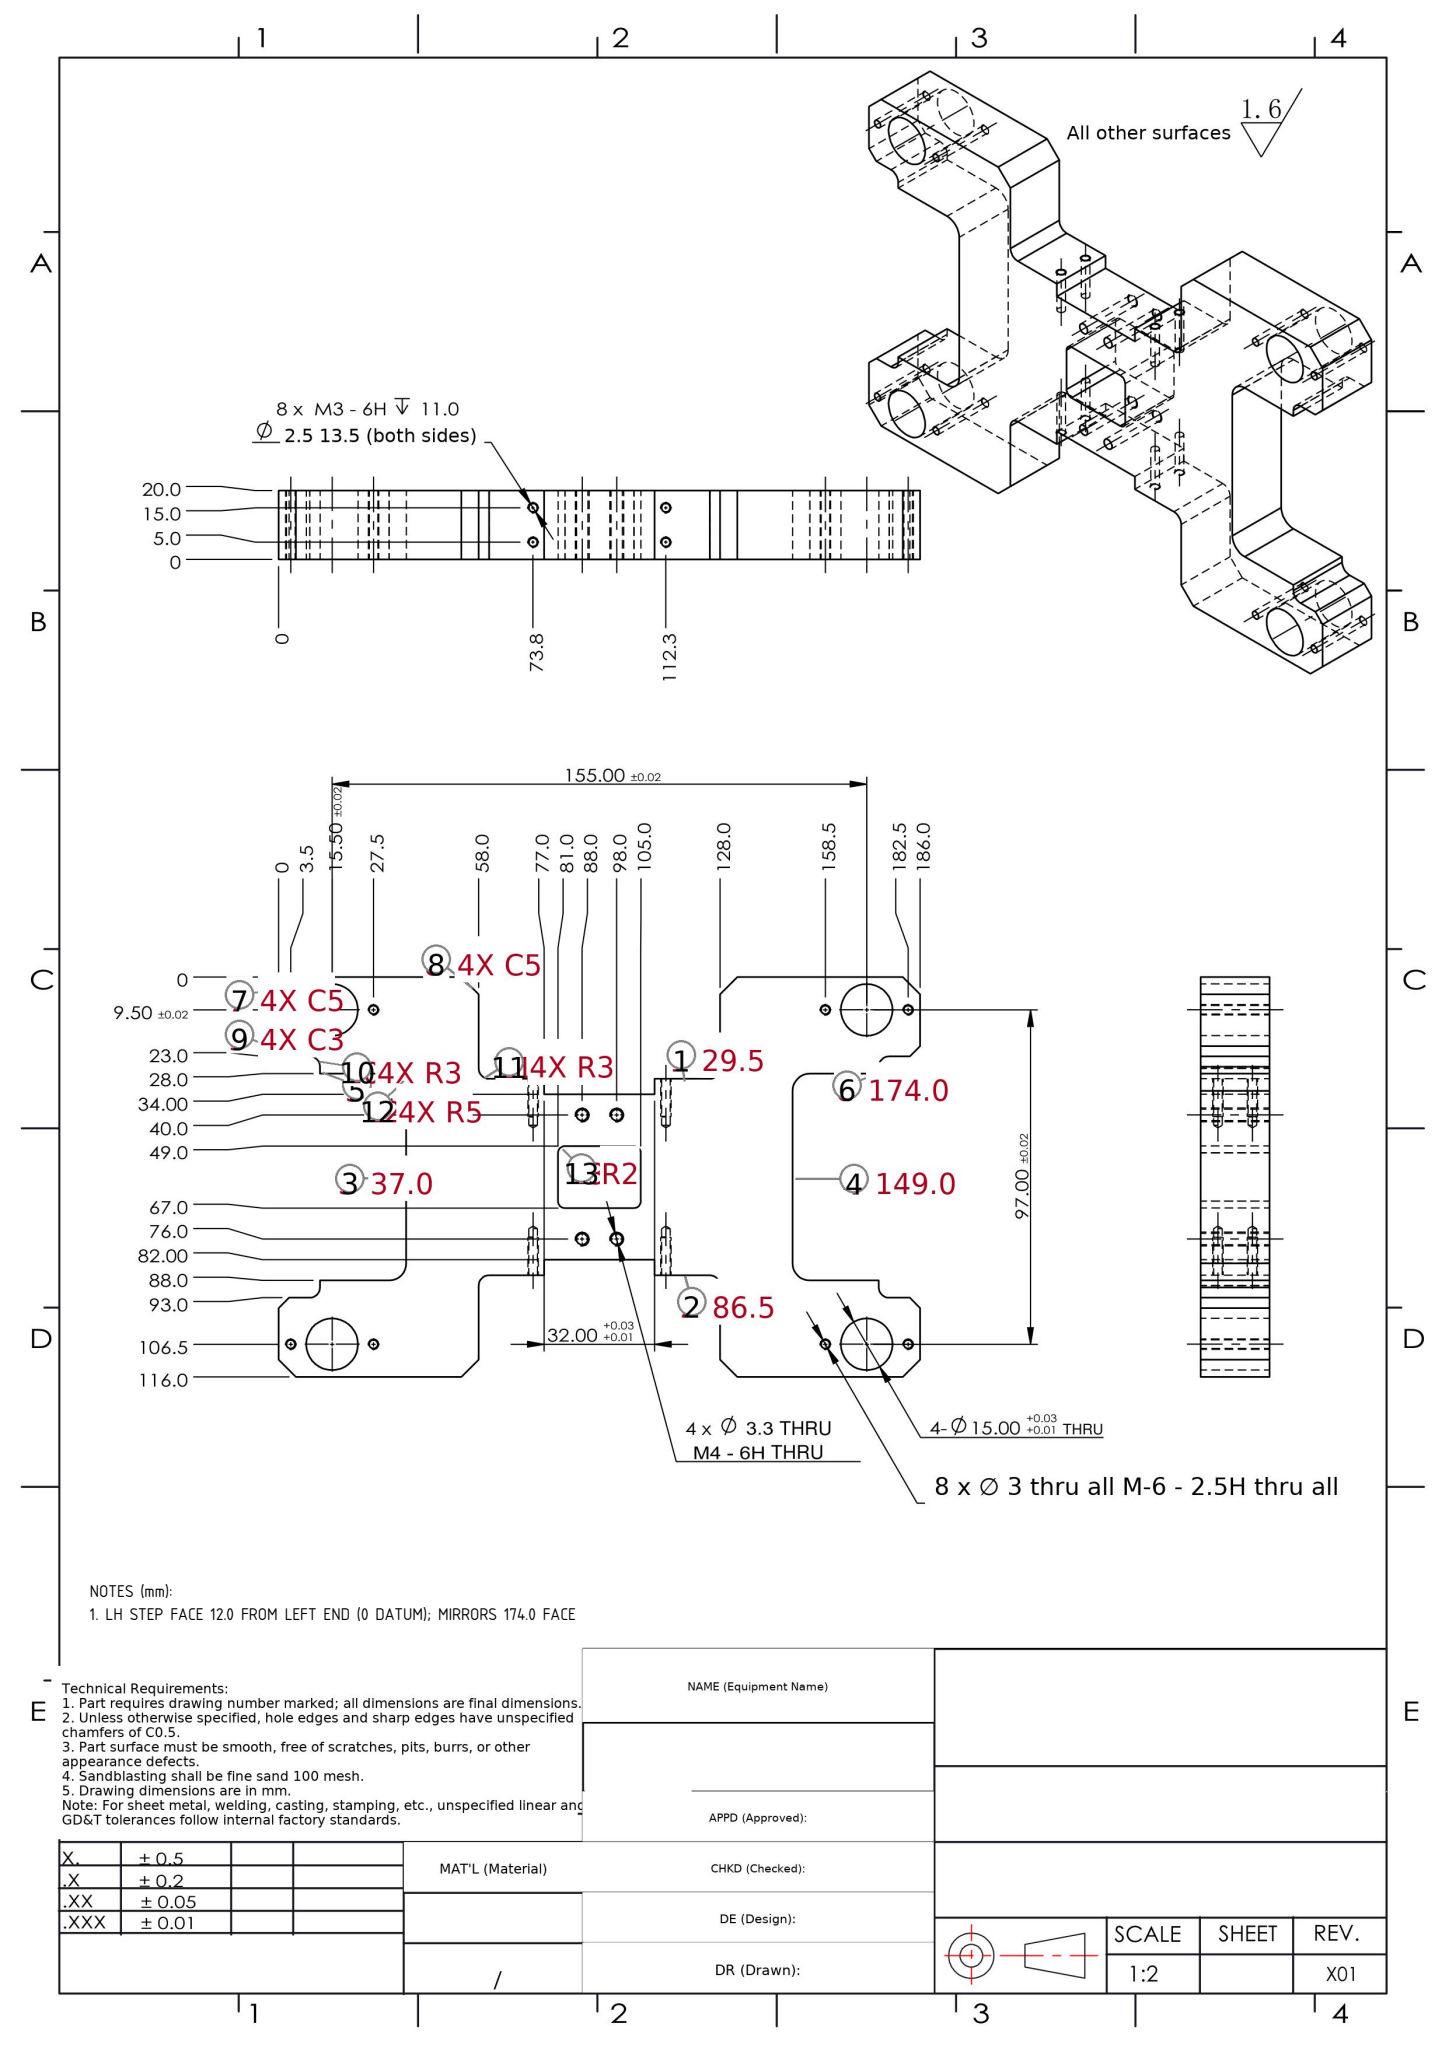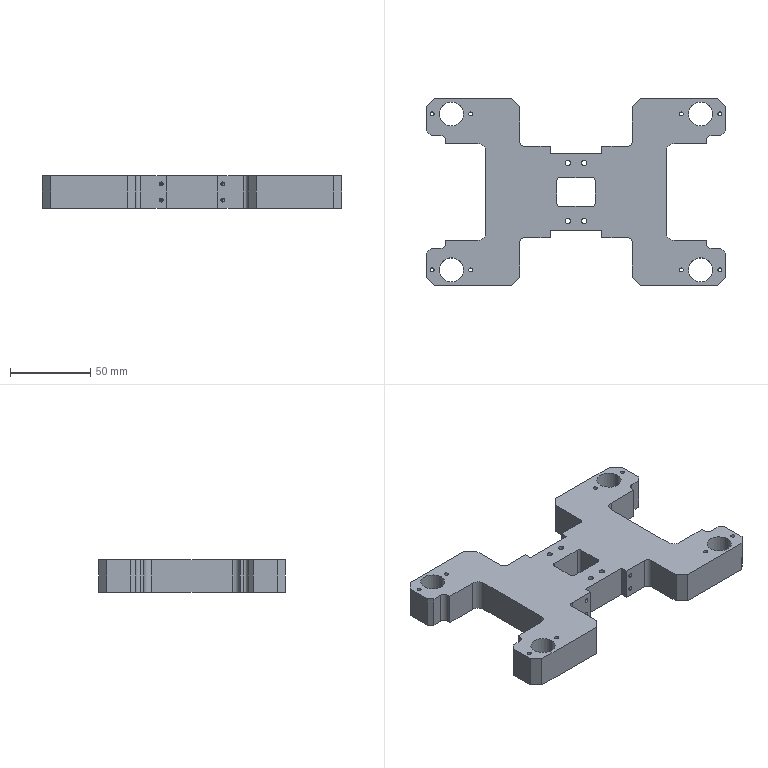Part | SolidWorks | mm | 1 solid | 134 faces | box 186 x 116 x 20 mm | volume 223220 mm3 | cylinder 64 | plane 54 | cone 16 | commonest cylinder face diameters 2.5 x32 3.3 x8 15 x8 6 x8 4 x4 10 x4
Drawing notes:
LH STEP FACE 12.0 FROM LEFT END (0 DATUM); MIRRORS 174.0 FACE | from the solid: axis_planes x=12.0 (2 faces), mirror of x=174.0 about bbox X=186.0 center
build123d program:
from build123d import *

# Parameters (mm, degrees)
SKETCH1_W                  = 190
SKETCH1_H                  = 130
BOSS_EXTRUDE1_DEPTH        = 20
SKETCH2_R                  = 7.5
CUT_EXTRUDE1_DEPTH         = 117.833
SKETCH6_W                  = 14
SKETCH6_H                  = 70
SKETCH6_W_2                = 70
SKETCH6_H_2                = 36.5
CUT_EXTRUDE5_DEPTH         = 117.833
CHAMFER1_SIZE              = 5
FILLET3_R                  = 3
M3_TAPPED_HOLE2_D          = 2.5
SKETCH28_W                 = 190
SKETCH28_H                 = 7
CUT_EXTRUDE11_DEPTH        = 117.833
SKETCH29_W                 = 2
SKETCH29_H                 = 116
CUT_EXTRUDE12_DEPTH        = 114.088
CHAMFER2_SIZE              = 5
SKETCH74_W                 = 32
SKETCH74_H                 = 4.5
CUT_EXTRUDE18_DEPTH        = 112.414
SKETCH75_W                 = 50
SKETCH75_H                 = 60
CUT_EXTRUDE19_DEPTH        = 112.414
M3_TAPPED_HOLE3_AT_2_COUNT = 2
M3_TAPPED_HOLE3_AT_2_PITCH = 10
M3_TAPPED_HOLE3_AT_3_COUNT = 2
M3_TAPPED_HOLE3_AT_3_PITCH = 38.5
M3_TAPPED_HOLE3_AT_4_COUNT = 2
M3_TAPPED_HOLE3_AT_4_PITCH = 39.778
SKETCH78_W                 = 24
SKETCH78_H                 = 18
CUT_EXTRUDE20_DEPTH        = 112.414
FILLET4_R                  = 2
M4_TAPPED_HOLE1_D          = 3.3
FILLET5_R                  = 5


with BuildPart() as part:
    # Sketch1 → Boss-Extrude1 (new body)
    with BuildSketch(Plane.XY):
        Rectangle(SKETCH1_W, SKETCH1_H)
    extrude(amount=BOSS_EXTRUDE1_DEPTH)

    # Sketch2 → Cut-Extrude1 (cut, through all)
    with BuildSketch(Plane.XY.offset(20)):
        with Locations((-77.5, 48.5)):
            Circle(SKETCH2_R)
        with Locations((-77.5, -48.5)):
            Circle(SKETCH2_R)
        with Locations((77.5, -48.5)):
            Circle(SKETCH2_R)
        with Locations((77.5, 48.5)):
            Circle(SKETCH2_R)
    extrude(amount=-CUT_EXTRUDE1_DEPTH, mode=Mode.SUBTRACT)

    # Sketch6 → Cut-Extrude5 (cut, through all)
    with BuildSketch(Plane(origin=(0, 0, 0), x_dir=(-1, 0, 0), z_dir=(0, 0, -1))):
        with Locations((-88, 0)):
            Rectangle(SKETCH6_W, SKETCH6_H)
        with Locations((0, 46.75)):
            Rectangle(SKETCH6_W_2, SKETCH6_H_2)
        with Locations((0, -46.75)):
            Rectangle(SKETCH6_W_2, SKETCH6_H_2)
        with Locations((88, 0)):
            Rectangle(SKETCH6_W, SKETCH6_H)
    extrude(amount=-CUT_EXTRUDE5_DEPTH, mode=Mode.SUBTRACT)

    # Chamfer1
    chamfer1_edges = [part.edges().sort_by_distance(p)[0] for p in [
        (95, -35, 10),
        (95, 35, 10),
        (35, 65, 10),
        (-35, 65, 10),
        (35, -65, 10),
        (-35, -65, 10),
        (95, -65, 10),
        (-95, -65, 10),
        (-95, 65, 10),
        (95, 65, 10),
        (-95, 35, 10),
        (-95, -35, 10),
    ]]
    chamfer(chamfer1_edges, length=CHAMFER1_SIZE)

    # Fillet3
    fillet3_edges = [part.edges().sort_by_distance(p)[0] for p in [
        (81, 35, 10),
        (81, -35, 10),
        (35, 28.5, 10),
        (-35, 28.5, 10),
        (35, -28.5, 10),
        (-35, -28.5, 10),
        (-81, -35, 10),
        (-81, 35, 10),
    ]]
    fillet(fillet3_edges, radius=FILLET3_R)

    # M3 Tapped Hole2 (through all)
    with Locations(Plane(origin=(0, 0, 0), x_dir=(-1, 0, 0), z_dir=(0, 0, -1))):
        with Locations((89.5, -48.5), (65.5, -48.5), (-65.5, -48.5), (-89.5, -48.5), (89.5, 48.5), (65.5, 48.5), (-65.5, 48.5), (-89.5, 48.5)):
            Hole(M3_TAPPED_HOLE2_D / 2)

    # Sketch28 → Cut-Extrude11 (cut, through all)
    with BuildSketch(Plane(origin=(0, 0, 0), x_dir=(-1, 0, 0), z_dir=(0, 0, -1))):
        with Locations((0, 61.5)):
            Rectangle(SKETCH28_W, SKETCH28_H)
        with Locations((0, -61.5)):
            Rectangle(SKETCH28_W, SKETCH28_H)
    extrude(amount=-CUT_EXTRUDE11_DEPTH, mode=Mode.SUBTRACT)

    # Sketch29 → Cut-Extrude12 (cut, through all)
    with BuildSketch(Plane(origin=(0, 0, 0), x_dir=(-1, 0, 0), z_dir=(0, 0, -1))):
        with Locations((-94, 0)):
            Rectangle(SKETCH29_W, SKETCH29_H)
        with Locations((94, 0)):
            Rectangle(SKETCH29_W, SKETCH29_H)
    extrude(amount=-CUT_EXTRUDE12_DEPTH, mode=Mode.SUBTRACT)

    # Chamfer2
    chamfer2_edges = [part.edges().sort_by_distance(p)[0] for p in [
        (-35, 58, 10),
        (35, 58, 10),
        (-35, -58, 10),
        (35, -58, 10),
        (93, 58, 10),
        (93, -58, 10),
        (-93, -58, 10),
        (-93, 58, 10),
    ]]
    chamfer(chamfer2_edges, length=CHAMFER2_SIZE)

    # Sketch74 → Cut-Extrude18 (cut, through all)
    with BuildSketch(Plane(origin=(0, 0, 0), x_dir=(-1, 0, 0), z_dir=(0, 0, -1))):
        with Locations((0, -26.25)):
            Rectangle(SKETCH74_W, SKETCH74_H)
        with Locations((0, 26.25)):
            Rectangle(SKETCH74_W, SKETCH74_H)
    extrude(amount=-CUT_EXTRUDE18_DEPTH, mode=Mode.SUBTRACT)

    # Sketch75 → Cut-Extrude19 (cut, through all)
    with BuildSketch(Plane.XY.offset(20)):
        with Locations((-81, 0)):
            Rectangle(SKETCH75_W, SKETCH75_H)
        with Locations((81, 0)):
            Rectangle(SKETCH75_W, SKETCH75_H)
    extrude(amount=-CUT_EXTRUDE19_DEPTH, mode=Mode.SUBTRACT)

    # Sketch76 → M3 Tapped Hole3 (revolve, cut)
    with BuildSketch(Plane(origin=(19.25, -28.5, 5), x_dir=(0, 0, -1), z_dir=(1, 0, 0))):
        Polygon((0, 0), (0, 14.251), (1.25, 13.5), (1.25, 0), align=None)
    m3_tapped_hole3 = revolve(axis=Axis((19.25, -34.85, 5), (0, 1, 0)), mode=Mode.SUBTRACT)

    # M3 Tapped Hole3 at 2: M3 Tapped Hole3 ×2
    with Locations(*[(0, 0, i * M3_TAPPED_HOLE3_AT_2_PITCH) for i in range(1, M3_TAPPED_HOLE3_AT_2_COUNT)]):
        add(m3_tapped_hole3, mode=Mode.SUBTRACT)

    # M3 Tapped Hole3 at 3: M3 Tapped Hole3 ×2
    with Locations(*[(-i * M3_TAPPED_HOLE3_AT_3_PITCH, 0, 0) for i in range(1, M3_TAPPED_HOLE3_AT_3_COUNT)]):
        add(m3_tapped_hole3, mode=Mode.SUBTRACT)

    # M3 Tapped Hole3 at 4: M3 Tapped Hole3 ×2
    with Locations(*[Vector(-0.9679, 0, 0.2514) * (i * M3_TAPPED_HOLE3_AT_4_PITCH) for i in range(1, M3_TAPPED_HOLE3_AT_4_COUNT)]):
        add(m3_tapped_hole3, mode=Mode.SUBTRACT)

    # Mirror1: M3 Tapped Hole3 across plane
    add(m3_tapped_hole3.mirror(Plane(origin=(0, 0, 0), x_dir=(0, 0, 1), z_dir=(0, -1, 0))), mode=Mode.SUBTRACT)

    # Mirror1 copy 1 sketch → Mirror1 copy 1 (revolve, cut)
    with BuildSketch(Plane(origin=(19.25, 28.5, 15), x_dir=(0, 0, -1), z_dir=(1, 0, 0))):
        Polygon((0, 0), (0, -14.251), (1.25, -13.5), (1.25, 0), align=None)
    revolve(axis=Axis((19.25, 34.85, 15), (0, 1, 0)), mode=Mode.SUBTRACT)

    # Mirror1 copy 2 sketch → Mirror1 copy 2 (revolve, cut)
    with BuildSketch(Plane(origin=(-19.25, 28.5, 5), x_dir=(0, 0, -1), z_dir=(1, 0, 0))):
        Polygon((0, 0), (0, -14.251), (1.25, -13.5), (1.25, 0), align=None)
    revolve(axis=Axis((-19.25, 34.85, 5), (0, 1, 0)), mode=Mode.SUBTRACT)

    # Mirror1 copy 3 sketch → Mirror1 copy 3 (revolve, cut)
    with BuildSketch(Plane(origin=(-19.25, 28.5, 15), x_dir=(0, 0, -1), z_dir=(1, 0, 0))):
        Polygon((0, 0), (0, -14.251), (1.25, -13.5), (1.25, 0), align=None)
    revolve(axis=Axis((-19.25, 34.85, 15), (0, 1, 0)), mode=Mode.SUBTRACT)

    # Sketch78 → Cut-Extrude20 (cut, through all)
    with BuildSketch(Plane(origin=(0, 0, 0), x_dir=(-1, 0, 0), z_dir=(0, 0, -1))):
        Rectangle(SKETCH78_W, SKETCH78_H)
    extrude(amount=-CUT_EXTRUDE20_DEPTH, mode=Mode.SUBTRACT)

    # Fillet4
    fillet4_edges = [part.edges().sort_by_distance(p)[0] for p in [
        (12, -9, 10),
        (12, 9, 10),
        (-12, 9, 10),
        (-12, -9, 10),
    ]]
    fillet(fillet4_edges, radius=FILLET4_R)

    # M4 Tapped Hole1 (through all)
    with Locations(Plane(origin=(0, 0, 0), x_dir=(-1, 0, 0), z_dir=(0, 0, -1))):
        with Locations((5, -18), (-5, -18), (5, 18), (-5, 18)):
            Hole(M4_TAPPED_HOLE1_D / 2)

    # Fillet5
    fillet5_edges = [part.edges().sort_by_distance(p)[0] for p in [
        (-56, -30, 10),
        (-56, 30, 10),
        (56, 30, 10),
        (56, -30, 10),
    ]]
    fillet(fillet5_edges, radius=FILLET5_R)


solid = part.part